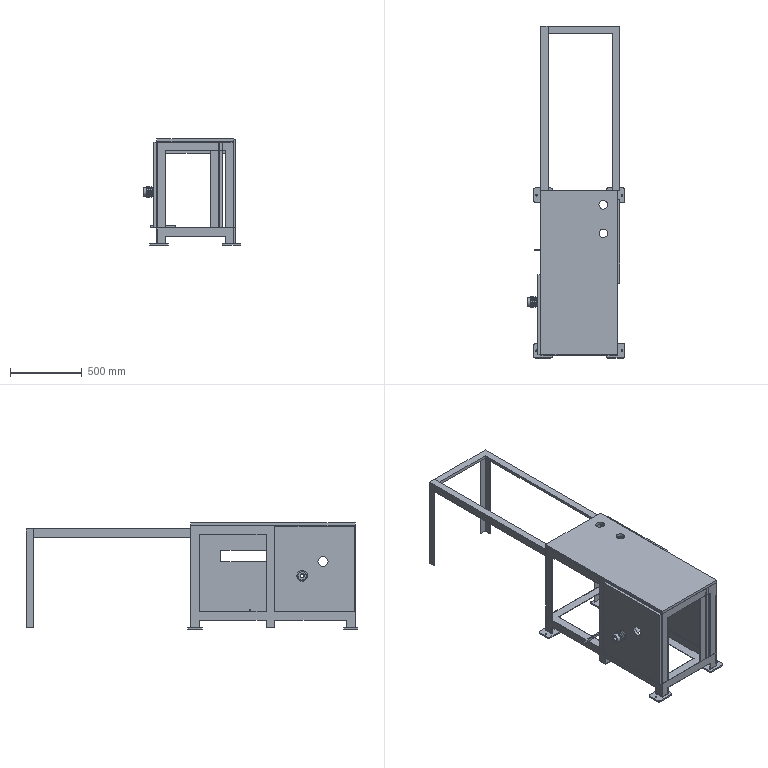Assembly | NX | mm | 7 component files | 8 solids | 246 faces | box 679.91 x 2313 x 741.5 mm | volume 39624236 mm3 | plane 204 | cylinder 36 | cone 6 | commonest cylinder face diameters 20 x16 70 x4 12.5 x4 58 x4 60 x2 10 x1 28 x1 73.01 x1
Bill of materials:
unnamed part 1 | 1 |  | Rectangular frame structure shaped like a table or stand: a solid flat top plate with two round through-holes near one end, held up by vertical square-section legs. Rectangular lower perimeter members tie the legs together, an intermediate pair of legs and a cross member sit part-way along the length, and small flat foot pads with small holes sit under the outer legs.
unnamed part 2 | 1 |  | Open frame made of slender square- or rectangular-section bar members: two parallel horizontal top rails joined by a cross rail at one end, with vertical posts hanging down from the corners at that end. It looks like an incomplete or partial frame weldment.
unnamed part 3 | 1 |  | Thin flat square plate with two round through-holes of similar size, placed diagonally offset from each other in the upper-central area.
unnamed part 4 | 1 |  | Thin flat square plate with two round through-holes of similar size, placed diagonally offset from each other in the upper-central area.
unnamed part 5 | 1 |  | Long straight prismatic bar with a rectangular cross-section. A small circular feature, possibly a hole or recess, shows faintly on one side face near the middle.
unnamed part 6 | 1 |  | Turned cylindrical part with three V-shaped circumferential grooves on its larger-diameter section and a smaller-diameter plain cylindrical hub sticking out from one side. A central round bore runs through it, with one keyway notch. It resembles a multi-groove sheave or pulley.
unnamed part 7 | 1 |  | Thin flat square plate with one rectangular through-slot, placed off-center toward the upper part of the plate.
Mates:
1. fix | Support_Bracket 1 component
2. touch align | Motor_Adjust_Plate 1 face | Support_Bracket 1 face